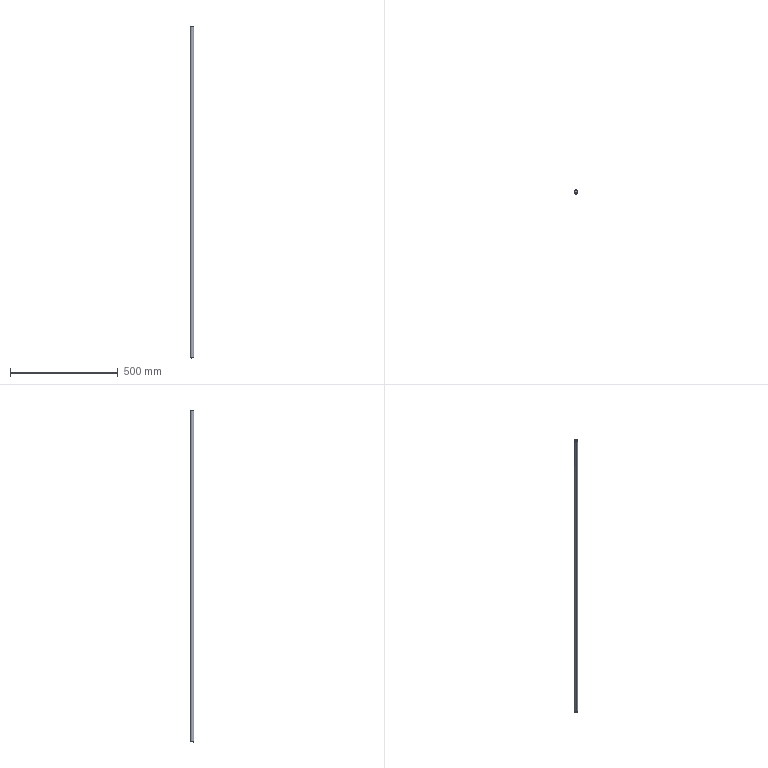Component | SolidWorks | Part19-1 | 1 solid | 8 faces | box 17 x 17 x 1540 mm | volume 349359 mm3 | torus 4 | cylinder 2 | plane 2 | commonest cylinder face diameters 17 x2
build123d program:
from build123d import *

# Parameters (mm, degrees)
SKETCH1_R           = 8.5
BOSS_EXTRUDE1_DEPTH = 1540
FILLET1_R           = 3
FILLET2_R           = 3


with BuildPart() as part:
    # Sketch1 → Boss-Extrude1 (new body)
    with BuildSketch(Plane.XY):
        Circle(SKETCH1_R)
    extrude(amount=BOSS_EXTRUDE1_DEPTH)

    # Fillet1
    fillet1_edges = [part.edges().sort_by_distance(p)[0] for p in [
        (-8.5, 0, 1540),
    ]]
    fillet(fillet1_edges, radius=FILLET1_R)

    # Fillet2
    fillet2_edges = [part.edges().sort_by_distance(p)[0] for p in [
        (-8.5, 0, 0),
    ]]
    fillet(fillet2_edges, radius=FILLET2_R)


solid = part.part

# Placed as in the assembly
solid = solid.moved(Location((231.081, -840.363, 1042.971), (0, 0, 0)))
STEP:
#1=COLOUR_RGB('',0.7922,0.8196,0.9333);
#2=FILL_AREA_STYLE_COLOUR('',#1);
#3=FILL_AREA_STYLE('',(#2));
#4=SURFACE_STYLE_FILL_AREA(#3);
#5=SURFACE_SIDE_STYLE('',(#4));
#6=SURFACE_STYLE_USAGE(.BOTH.,#5);
#7=PRESENTATION_STYLE_ASSIGNMENT((#6));
#8=CARTESIAN_POINT('',(8.981,-33.267,41.062));
#9=VERTEX_POINT('',#8);
#10=CARTESIAN_POINT('',(9.215,-32.903,41.062));
#11=VERTEX_POINT('',#10);
#12=CARTESIAN_POINT('',(9.098,-33.085,41.062));
#13=DIRECTION('',(0.,0.,-1.));
#14=DIRECTION('',(0.5403,0.8415,0.));
#15=AXIS2_PLACEMENT_3D('',#12,#13,#14);
#16=CIRCLE('',#15,0.2165);
#17=EDGE_CURVE('',#9,#11,#16,.T.);
#18=ORIENTED_EDGE('',*,*,#17,.F.);
#19=CARTESIAN_POINT('',(8.917,-33.367,41.18));
#20=VERTEX_POINT('',#19);
#21=CARTESIAN_POINT('',(8.981,-33.267,41.18));
#22=DIRECTION('',(-0.8415,0.5403,0.));
#23=DIRECTION('',(-0.5403,-0.8415,0.));
#24=AXIS2_PLACEMENT_3D('',#21,#22,#23);
#25=CIRCLE('',#24,0.1181);
#26=EDGE_CURVE('',#9,#20,#25,.T.);
#27=ORIENTED_EDGE('',*,*,#26,.T.);
#28=CARTESIAN_POINT('',(9.278,-32.804,41.18));
#29=VERTEX_POINT('',#28);
#30=CARTESIAN_POINT('',(9.098,-33.085,41.18));
#31=DIRECTION('',(-0.,-0.,1.));
#32=DIRECTION('',(0.5403,0.8415,0.));
#33=AXIS2_PLACEMENT_3D('',#30,#31,#32);
#34=CIRCLE('',#33,0.3346);
#35=EDGE_CURVE('',#29,#20,#34,.T.);
#36=ORIENTED_EDGE('',*,*,#35,.F.);
#37=CARTESIAN_POINT('',(9.215,-32.903,41.18));
#38=DIRECTION('',(0.8415,-0.5403,-0.));
#39=DIRECTION('',(0.5403,0.8415,0.));
#40=AXIS2_PLACEMENT_3D('',#37,#38,#39);
#41=CIRCLE('',#40,0.1181);
#42=EDGE_CURVE('',#11,#29,#41,.T.);
#43=ORIENTED_EDGE('',*,*,#42,.F.);
#44=EDGE_LOOP('',(#18,#27,#36,#43));
#45=FACE_OUTER_BOUND('',#44,.T.);
#46=CARTESIAN_POINT('',(9.098,-33.085,41.18));
#47=DIRECTION('',(-0.,-0.,1.));
#48=DIRECTION('',(0.5403,0.8415,0.));
#49=AXIS2_PLACEMENT_3D('',#46,#47,#48);
#50=TOROIDAL_SURFACE('',#49,0.2165,0.1181);
#51=ADVANCED_FACE('',(#45),#50,.T.);
#52=CARTESIAN_POINT('',(8.917,-33.367,101.574));
#53=VERTEX_POINT('',#52);
#54=CARTESIAN_POINT('',(9.278,-32.804,101.574));
#55=VERTEX_POINT('',#54);
#56=CARTESIAN_POINT('',(9.098,-33.085,101.574));
#57=DIRECTION('',(0.,0.,-1.));
#58=DIRECTION('',(0.5403,0.8415,0.));
#59=AXIS2_PLACEMENT_3D('',#56,#57,#58);
#60=CIRCLE('',#59,0.3346);
#61=EDGE_CURVE('',#53,#55,#60,.T.);
#62=ORIENTED_EDGE('',*,*,#61,.F.);
#63=CARTESIAN_POINT('',(8.981,-33.267,101.692));
#64=VERTEX_POINT('',#63);
#65=CARTESIAN_POINT('',(8.981,-33.267,101.574));
#66=DIRECTION('',(-0.8415,0.5403,0.));
#67=DIRECTION('',(-0.5403,-0.8415,0.));
#68=AXIS2_PLACEMENT_3D('',#65,#66,#67);
#69=CIRCLE('',#68,0.1181);
#70=EDGE_CURVE('',#53,#64,#69,.T.);
#71=ORIENTED_EDGE('',*,*,#70,.T.);
#72=CARTESIAN_POINT('',(9.215,-32.903,101.692));
#73=VERTEX_POINT('',#72);
#74=CARTESIAN_POINT('',(9.098,-33.085,101.692));
#75=DIRECTION('',(-0.,-0.,1.));
#76=DIRECTION('',(0.5403,0.8415,0.));
#77=AXIS2_PLACEMENT_3D('',#74,#75,#76);
#78=CIRCLE('',#77,0.2165);
#79=EDGE_CURVE('',#73,#64,#78,.T.);
#80=ORIENTED_EDGE('',*,*,#79,.F.);
#81=CARTESIAN_POINT('',(9.215,-32.903,101.574));
#82=DIRECTION('',(0.8415,-0.5403,-0.));
#83=DIRECTION('',(0.5403,0.8415,0.));
#84=AXIS2_PLACEMENT_3D('',#81,#82,#83);
#85=CIRCLE('',#84,0.1181);
#86=EDGE_CURVE('',#55,#73,#85,.T.);
#87=ORIENTED_EDGE('',*,*,#86,.F.);
#88=EDGE_LOOP('',(#62,#71,#80,#87));
#89=FACE_OUTER_BOUND('',#88,.T.);
#90=CARTESIAN_POINT('',(9.098,-33.085,101.574));
#91=DIRECTION('',(-0.,-0.,1.));
#92=DIRECTION('',(0.5403,0.8415,0.));
#93=AXIS2_PLACEMENT_3D('',#90,#91,#92);
#94=TOROIDAL_SURFACE('',#93,0.2165,0.1181);
#95=ADVANCED_FACE('',(#89),#94,.T.);
#96=ORIENTED_EDGE('',*,*,#61,.T.);
#97=CARTESIAN_POINT('',(9.278,-32.804,101.692));
#98=DIRECTION('',(0.,0.,-1.));
#99=VECTOR('',#98,39.37);
#100=LINE('',#97,#99);
#101=EDGE_CURVE('',#55,#29,#100,.T.);
#102=ORIENTED_EDGE('',*,*,#101,.T.);
#103=ORIENTED_EDGE('',*,*,#35,.T.);
#104=CARTESIAN_POINT('',(8.917,-33.367,101.692));
#105=DIRECTION('',(0.,0.,-1.));
#106=VECTOR('',#105,39.37);
#107=LINE('',#104,#106);
#108=EDGE_CURVE('',#53,#20,#107,.T.);
#109=ORIENTED_EDGE('',*,*,#108,.F.);
#110=EDGE_LOOP('',(#96,#102,#103,#109));
#111=FACE_OUTER_BOUND('',#110,.T.);
#112=CARTESIAN_POINT('',(9.098,-33.085,101.692));
#113=DIRECTION('',(0.,0.,-1.));
#114=DIRECTION('',(-0.5403,-0.8415,-0.));
#115=AXIS2_PLACEMENT_3D('',#112,#113,#114);
#116=CYLINDRICAL_SURFACE('',#115,0.3346);
#117=ADVANCED_FACE('',(#111),#116,.T.);
#118=ORIENTED_EDGE('',*,*,#101,.F.);
#119=CARTESIAN_POINT('',(9.098,-33.085,101.574));
#120=DIRECTION('',(0.,0.,-1.));
#121=DIRECTION('',(0.5403,0.8415,0.));
#122=AXIS2_PLACEMENT_3D('',#119,#120,#121);
#123=CIRCLE('',#122,0.3346);
#124=EDGE_CURVE('',#55,#53,#123,.T.);
#125=ORIENTED_EDGE('',*,*,#124,.T.);
#126=ORIENTED_EDGE('',*,*,#108,.T.);
#127=CARTESIAN_POINT('',(9.098,-33.085,41.18));
#128=DIRECTION('',(-0.,-0.,1.));
#129=DIRECTION('',(0.5403,0.8415,0.));
#130=AXIS2_PLACEMENT_3D('',#127,#128,#129);
#131=CIRCLE('',#130,0.3346);
#132=EDGE_CURVE('',#20,#29,#131,.T.);
#133=ORIENTED_EDGE('',*,*,#132,.T.);
#134=EDGE_LOOP('',(#118,#125,#126,#133));
#135=FACE_OUTER_BOUND('',#134,.T.);
#136=CARTESIAN_POINT('',(9.098,-33.085,101.692));
#137=DIRECTION('',(0.,0.,-1.));
#138=DIRECTION('',(-0.5403,-0.8415,-0.));
#139=AXIS2_PLACEMENT_3D('',#136,#137,#138);
#140=CYLINDRICAL_SURFACE('',#139,0.3346);
#141=ADVANCED_FACE('',(#135),#140,.T.);
#142=ORIENTED_EDGE('',*,*,#79,.T.);
#143=CARTESIAN_POINT('',(9.098,-33.085,101.692));
#144=DIRECTION('',(-0.,-0.,1.));
#145=DIRECTION('',(0.5403,0.8415,0.));
#146=AXIS2_PLACEMENT_3D('',#143,#144,#145);
#147=CIRCLE('',#146,0.2165);
#148=EDGE_CURVE('',#64,#73,#147,.T.);
#149=ORIENTED_EDGE('',*,*,#148,.T.);
#150=EDGE_LOOP('',(#142,#149));
#151=FACE_OUTER_BOUND('',#150,.T.);
#152=CARTESIAN_POINT('',(9.098,-33.085,101.692));
#153=DIRECTION('',(-0.,-0.,1.));
#154=DIRECTION('',(0.5403,0.8415,0.));
#155=AXIS2_PLACEMENT_3D('',#152,#153,#154);
#156=PLANE('',#155);
#157=ADVANCED_FACE('',(#151),#156,.T.);
#158=CARTESIAN_POINT('',(9.098,-33.085,41.062));
#159=DIRECTION('',(0.,0.,-1.));
#160=DIRECTION('',(0.5403,0.8415,0.));
#161=AXIS2_PLACEMENT_3D('',#158,#159,#160);
#162=CIRCLE('',#161,0.2165);
#163=EDGE_CURVE('',#11,#9,#162,.T.);
#164=ORIENTED_EDGE('',*,*,#163,.T.);
#165=ORIENTED_EDGE('',*,*,#17,.T.);
#166=EDGE_LOOP('',(#164,#165));
#167=FACE_OUTER_BOUND('',#166,.T.);
#168=CARTESIAN_POINT('',(9.098,-33.085,41.062));
#169=DIRECTION('',(-0.,-0.,1.));
#170=DIRECTION('',(0.5403,0.8415,0.));
#171=AXIS2_PLACEMENT_3D('',#168,#169,#170);
#172=PLANE('',#171);
#173=ADVANCED_FACE('',(#167),#172,.F.);
#174=ORIENTED_EDGE('',*,*,#70,.F.);
#175=ORIENTED_EDGE('',*,*,#124,.F.);
#176=ORIENTED_EDGE('',*,*,#86,.T.);
#177=ORIENTED_EDGE('',*,*,#148,.F.);
#178=EDGE_LOOP('',(#174,#175,#176,#177));
#179=FACE_OUTER_BOUND('',#178,.T.);
#180=CARTESIAN_POINT('',(9.098,-33.085,101.574));
#181=DIRECTION('',(-0.,-0.,1.));
#182=DIRECTION('',(0.5403,0.8415,0.));
#183=AXIS2_PLACEMENT_3D('',#180,#181,#182);
#184=TOROIDAL_SURFACE('',#183,0.2165,0.1181);
#185=ADVANCED_FACE('',(#179),#184,.T.);
#186=ORIENTED_EDGE('',*,*,#26,.F.);
#187=ORIENTED_EDGE('',*,*,#163,.F.);
#188=ORIENTED_EDGE('',*,*,#42,.T.);
#189=ORIENTED_EDGE('',*,*,#132,.F.);
#190=EDGE_LOOP('',(#186,#187,#188,#189));
#191=FACE_OUTER_BOUND('',#190,.T.);
#192=CARTESIAN_POINT('',(9.098,-33.085,41.18));
#193=DIRECTION('',(-0.,-0.,1.));
#194=DIRECTION('',(0.5403,0.8415,0.));
#195=AXIS2_PLACEMENT_3D('',#192,#193,#194);
#196=TOROIDAL_SURFACE('',#195,0.2165,0.1181);
#197=ADVANCED_FACE('',(#191),#196,.T.);
#198=CLOSED_SHELL('',(#51,#95,#117,#141,#157,#173,#185,#197));
#199=MANIFOLD_SOLID_BREP('',#198);
#200=STYLED_ITEM('',(#7),#199);
#201=(LENGTH_UNIT()NAMED_UNIT(*)SI_UNIT($,.METRE.));
#202=LENGTH_MEASURE_WITH_UNIT(LENGTH_MEASURE(0.0254),#201);
#203=DIMENSIONAL_EXPONENTS(1.,0.,0.,0.,0.,0.,0.);
#204=(CONVERSION_BASED_UNIT('',#202)LENGTH_UNIT()NAMED_UNIT(#203));
#205=UNCERTAINTY_MEASURE_WITH_UNIT(LENGTH_MEASURE(0.00001),#204,'','');
#206=(NAMED_UNIT(*)PLANE_ANGLE_UNIT()SI_UNIT($,.RADIAN.));
#207=(NAMED_UNIT(*)SI_UNIT($,.STERADIAN.)SOLID_ANGLE_UNIT());
#208=(GEOMETRIC_REPRESENTATION_CONTEXT(3)GLOBAL_UNCERTAINTY_ASSIGNED_CONTEXT((#205))GLOBAL_UNIT_ASSIGNED_CONTEXT((#204,#206,#207))REPRESENTATION_CONTEXT('',''));
#209=MECHANICAL_DESIGN_GEOMETRIC_PRESENTATION_REPRESENTATION('',(#200),#208);
#210=CARTESIAN_POINT('',(0.,0.,0.));
#211=DIRECTION('',(0.,0.,1.));
#212=DIRECTION('',(1.,0.,0.));
#213=AXIS2_PLACEMENT_3D('',#210,#211,#212);
#214=(LENGTH_UNIT()NAMED_UNIT(*)SI_UNIT($,.METRE.));
#215=LENGTH_MEASURE_WITH_UNIT(LENGTH_MEASURE(0.0254),#214);
#216=DIMENSIONAL_EXPONENTS(1.,0.,0.,0.,0.,0.,0.);
#217=(CONVERSION_BASED_UNIT('',#215)LENGTH_UNIT()NAMED_UNIT(#216));
#218=UNCERTAINTY_MEASURE_WITH_UNIT(LENGTH_MEASURE(0.00001),#217,'','');
#219=(NAMED_UNIT(*)PLANE_ANGLE_UNIT()SI_UNIT($,.RADIAN.));
#220=(NAMED_UNIT(*)SI_UNIT($,.STERADIAN.)SOLID_ANGLE_UNIT());
#221=(GEOMETRIC_REPRESENTATION_CONTEXT(3)GLOBAL_UNCERTAINTY_ASSIGNED_CONTEXT((#218))GLOBAL_UNIT_ASSIGNED_CONTEXT((#217,#219,#220))REPRESENTATION_CONTEXT('',''));
#222=ADVANCED_BREP_SHAPE_REPRESENTATION('',(#199,#213),#221);
#223=PRESENTATION_LAYER_ASSIGNMENT('','',(#200));